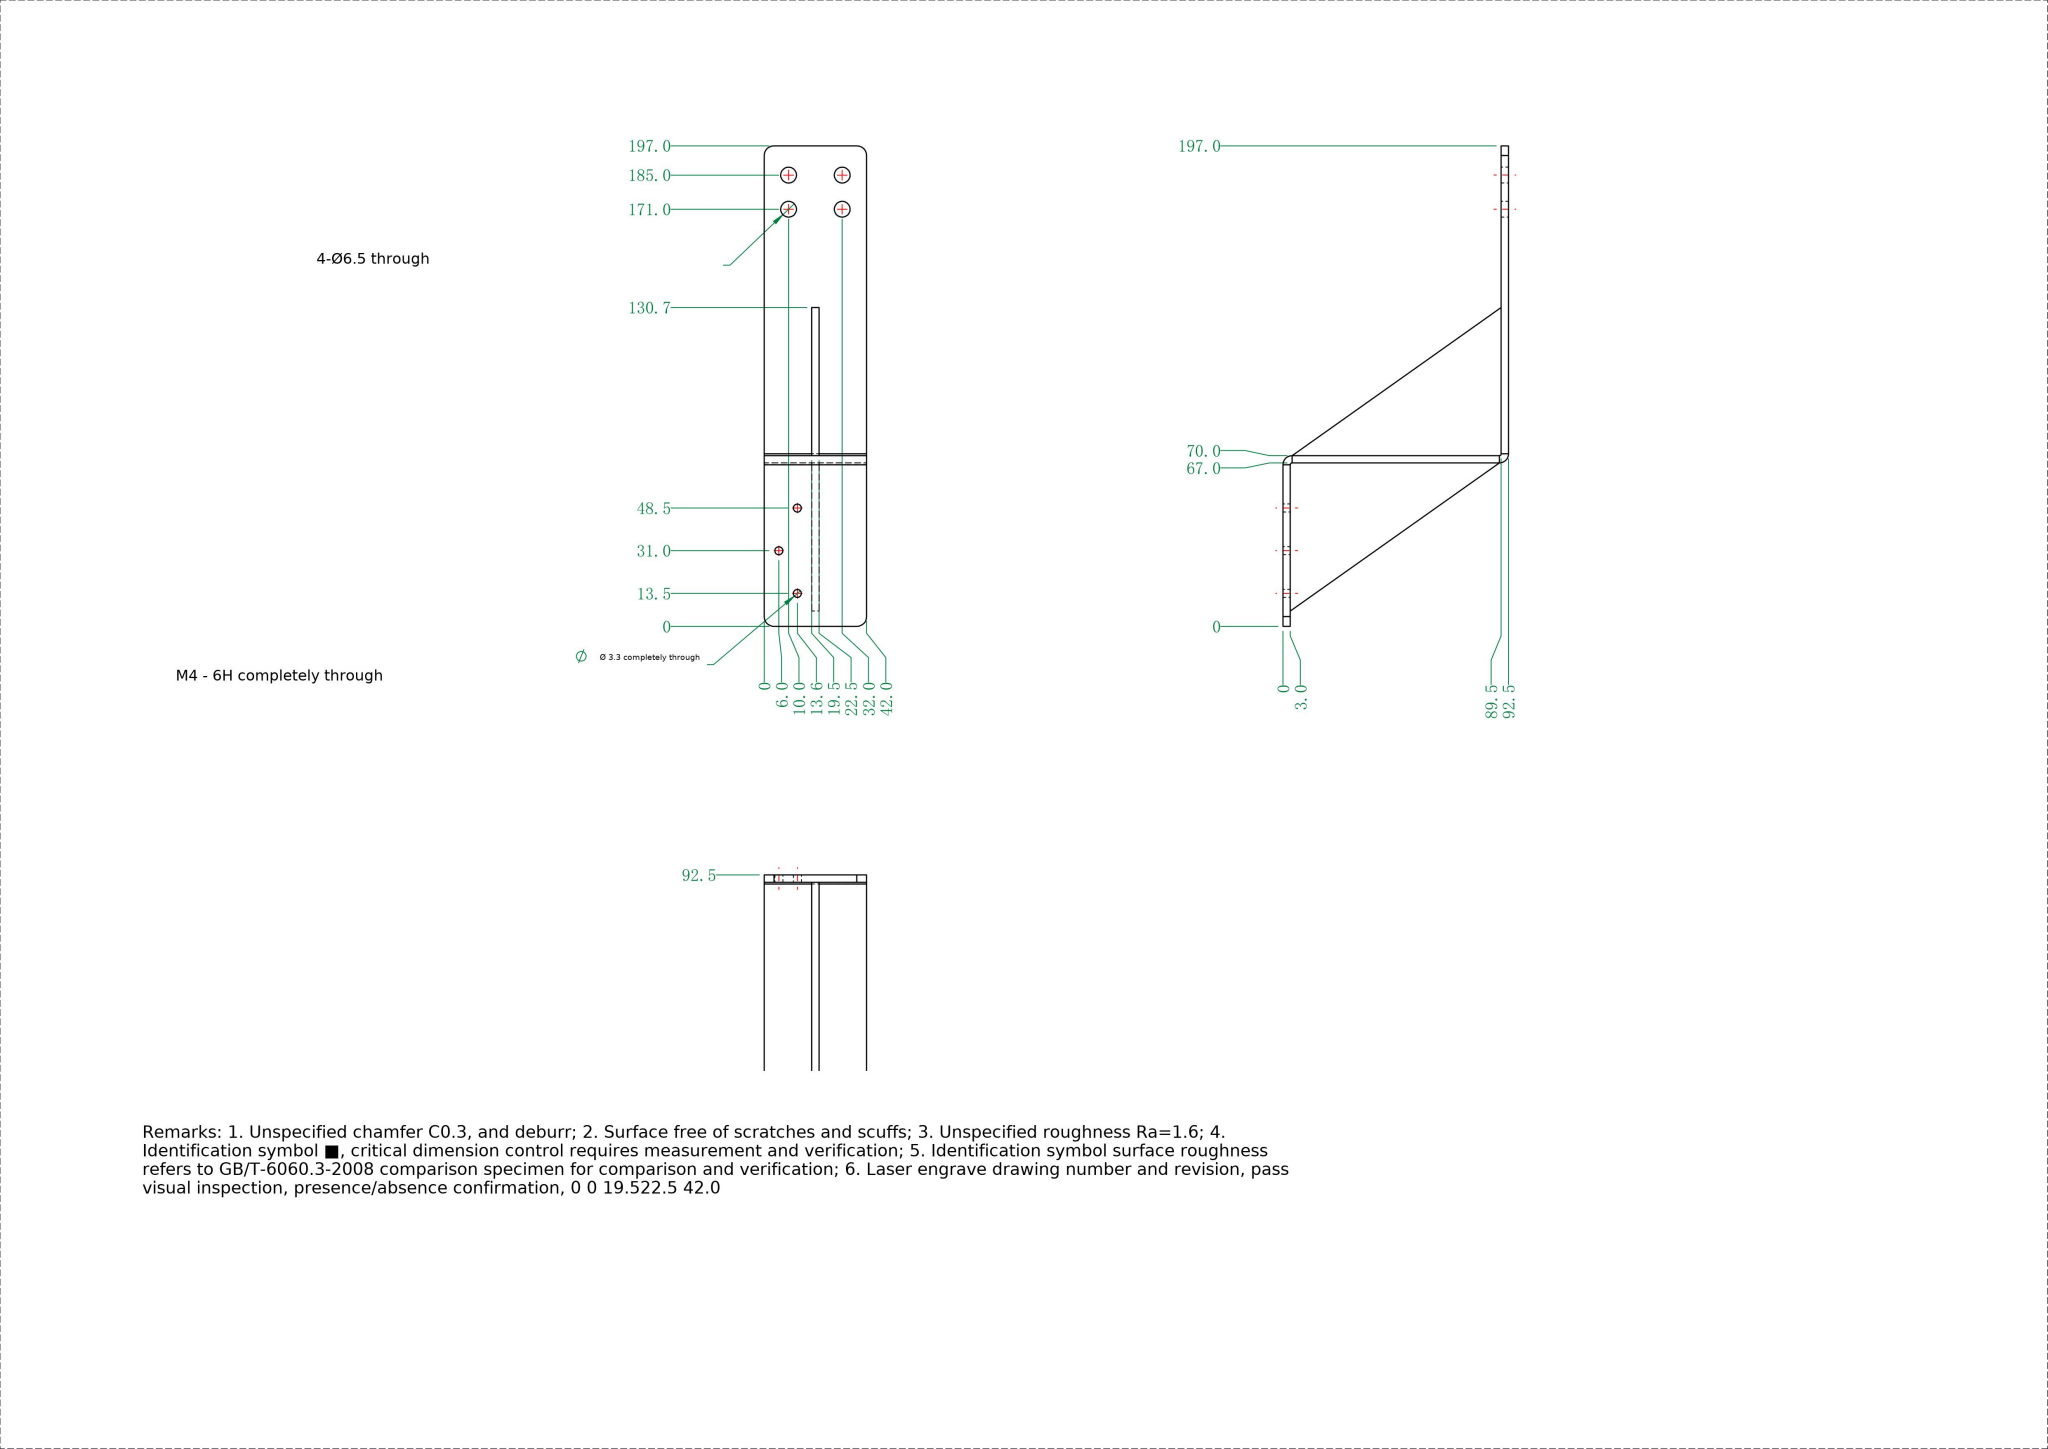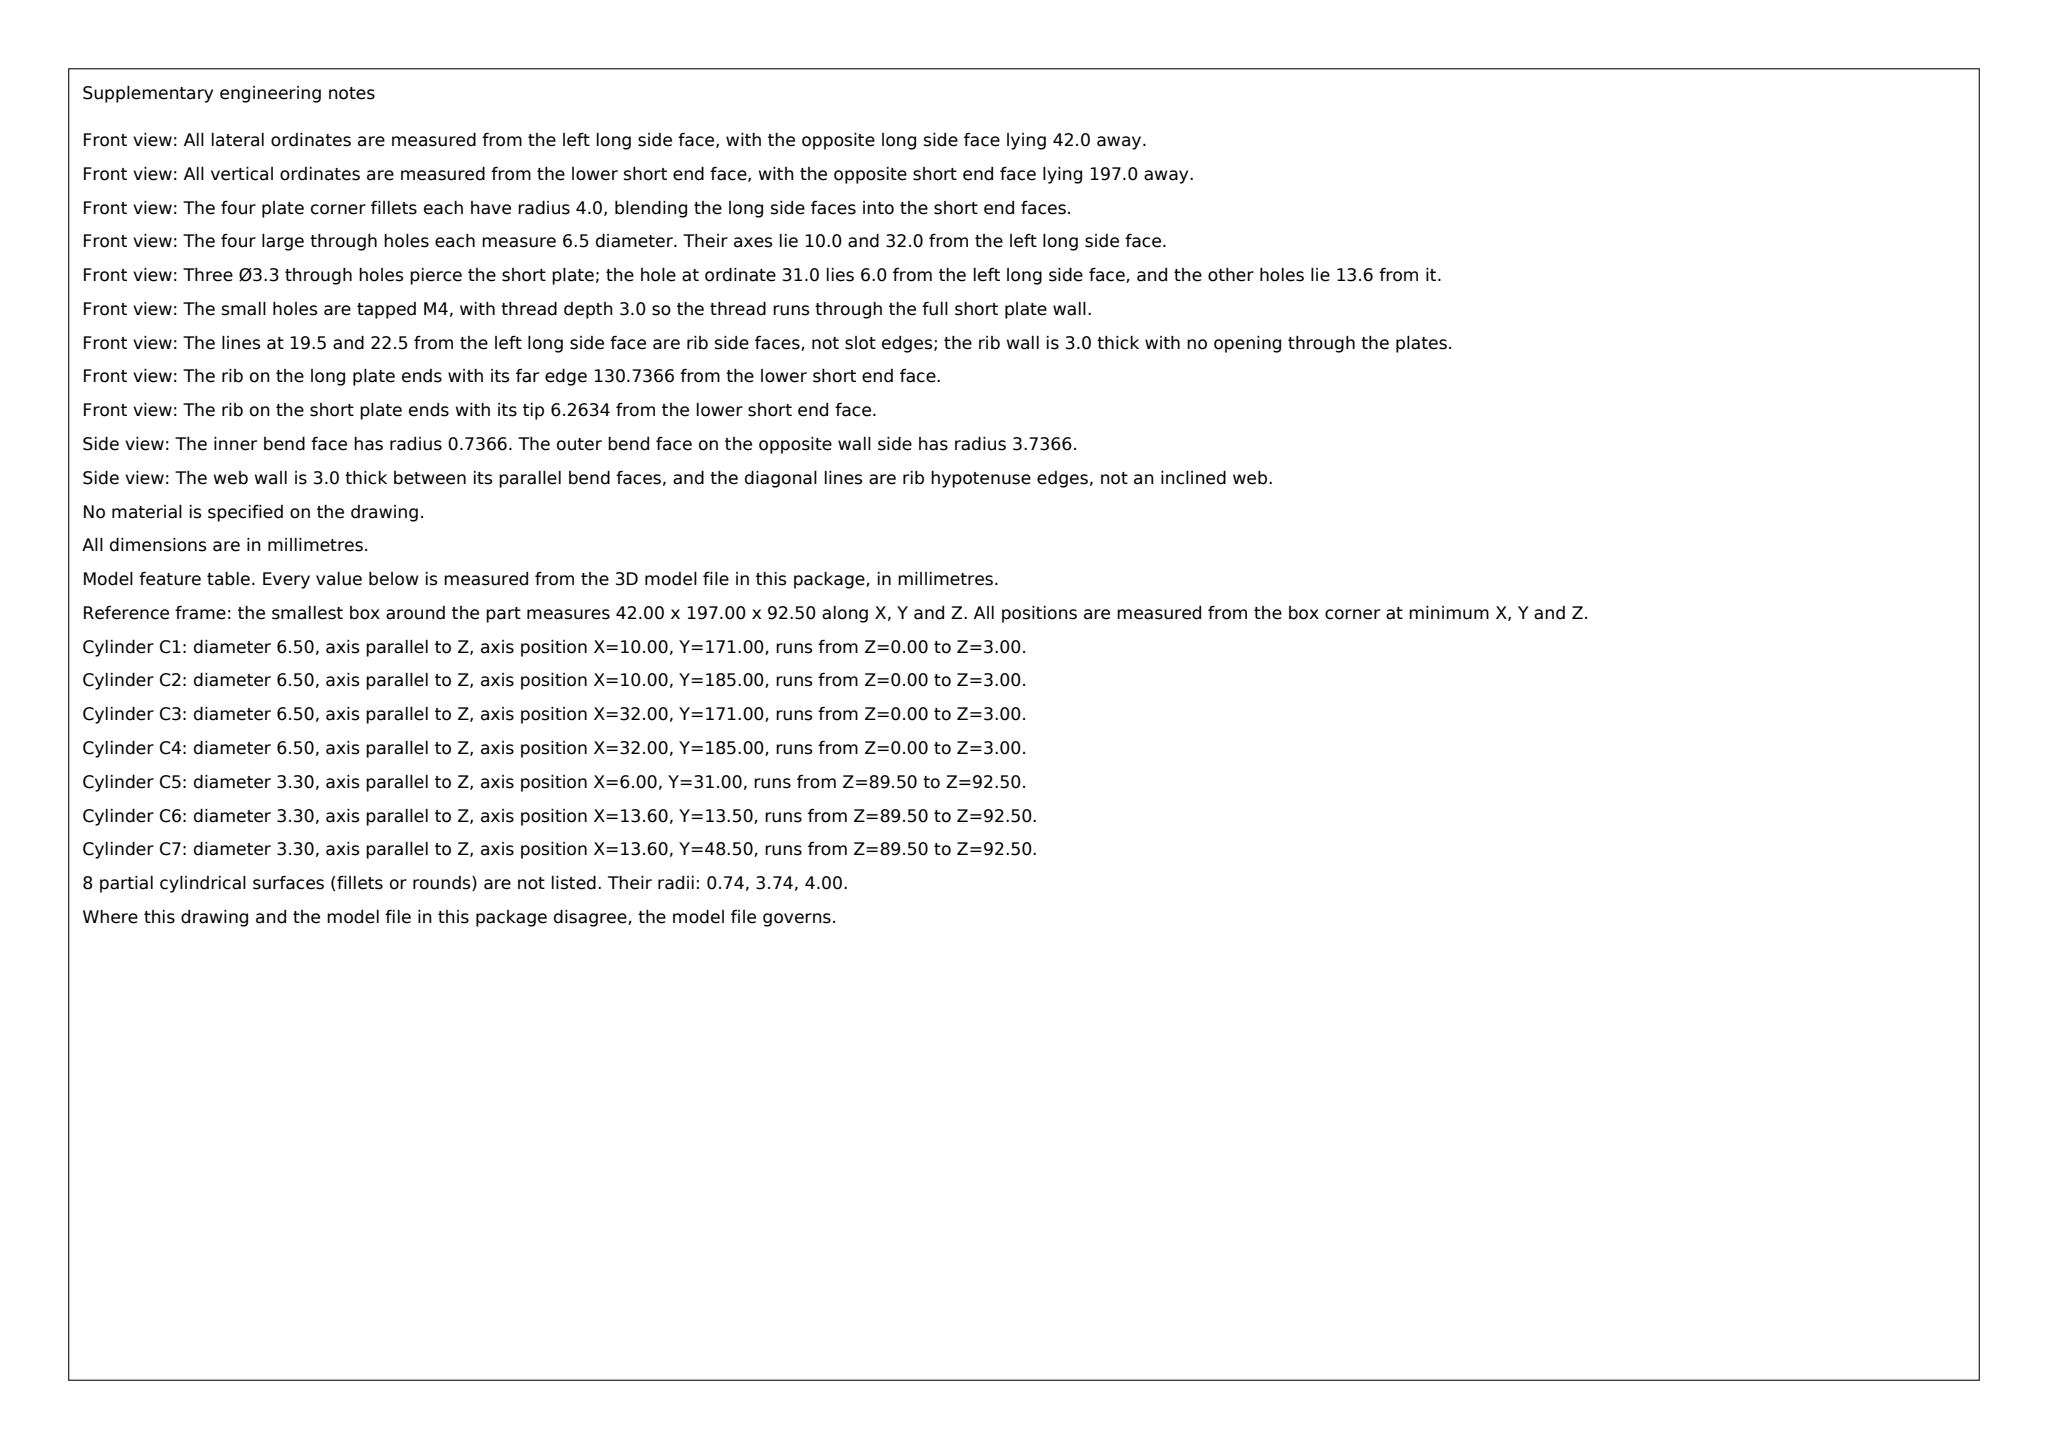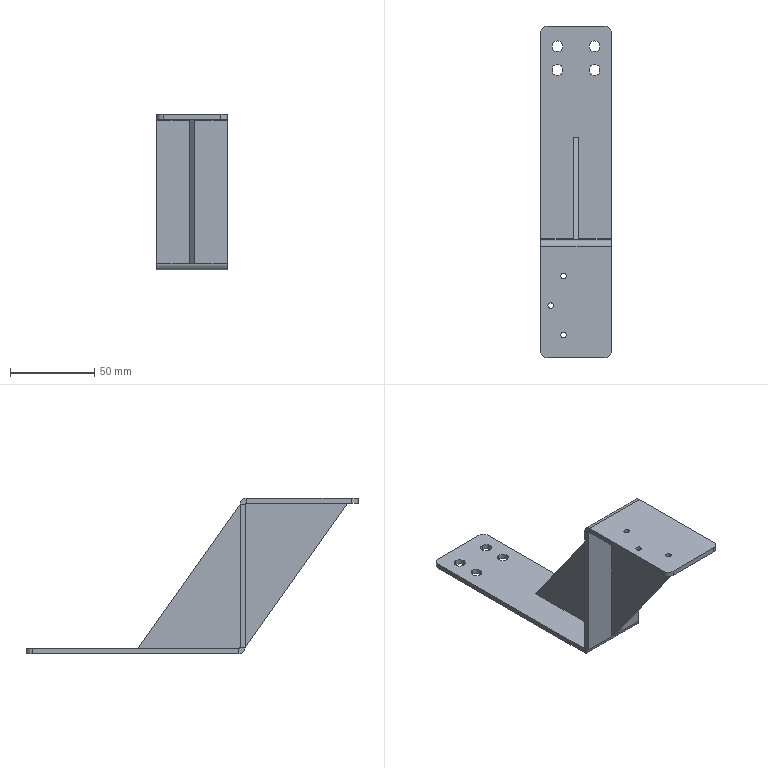Part | SolidWorks | mm | 1 solid | 50 faces | box 42 x 197 x 92.5 mm | volume 50967 mm3 | plane 26 | cylinder 24 | commonest cylinder face diameters 6.5 x8 3.3 x6 1.473 x4 8 x4 7.473 x2
Drawing notes:
3X M4-6H THRU AT X6.0/Y31.0, X13.6/Y13.5, X13.6/Y48.5 FROM LH EDGE | from the solid: Ø3.3 z-axis cyls at (6.0,31.0),(13.6,13.5),(13.6,48.5), len 3.0 = M4 tap drill
SLOT 3.0 WIDE (X19.5-X22.5) THRU, Y130.7 TO OPEN END Y0, CROSSES BEND | from the solid: x-normal planes at 19.5 & 22.5 (2 ea, plate + bent leg); bend cyls Ø1.473/7.473 split into 19.5 segs; no closed slot end plane at Y0
2-R0.7 INSIDE BEND RAD (BOTH BENDS) | from the solid: x-axis cyls dia 1.473 at y66.26/z88.76 and y70.74/z3.74 -> inside R0.7365; outer dia 7.473 = R0.7+3.0 thk